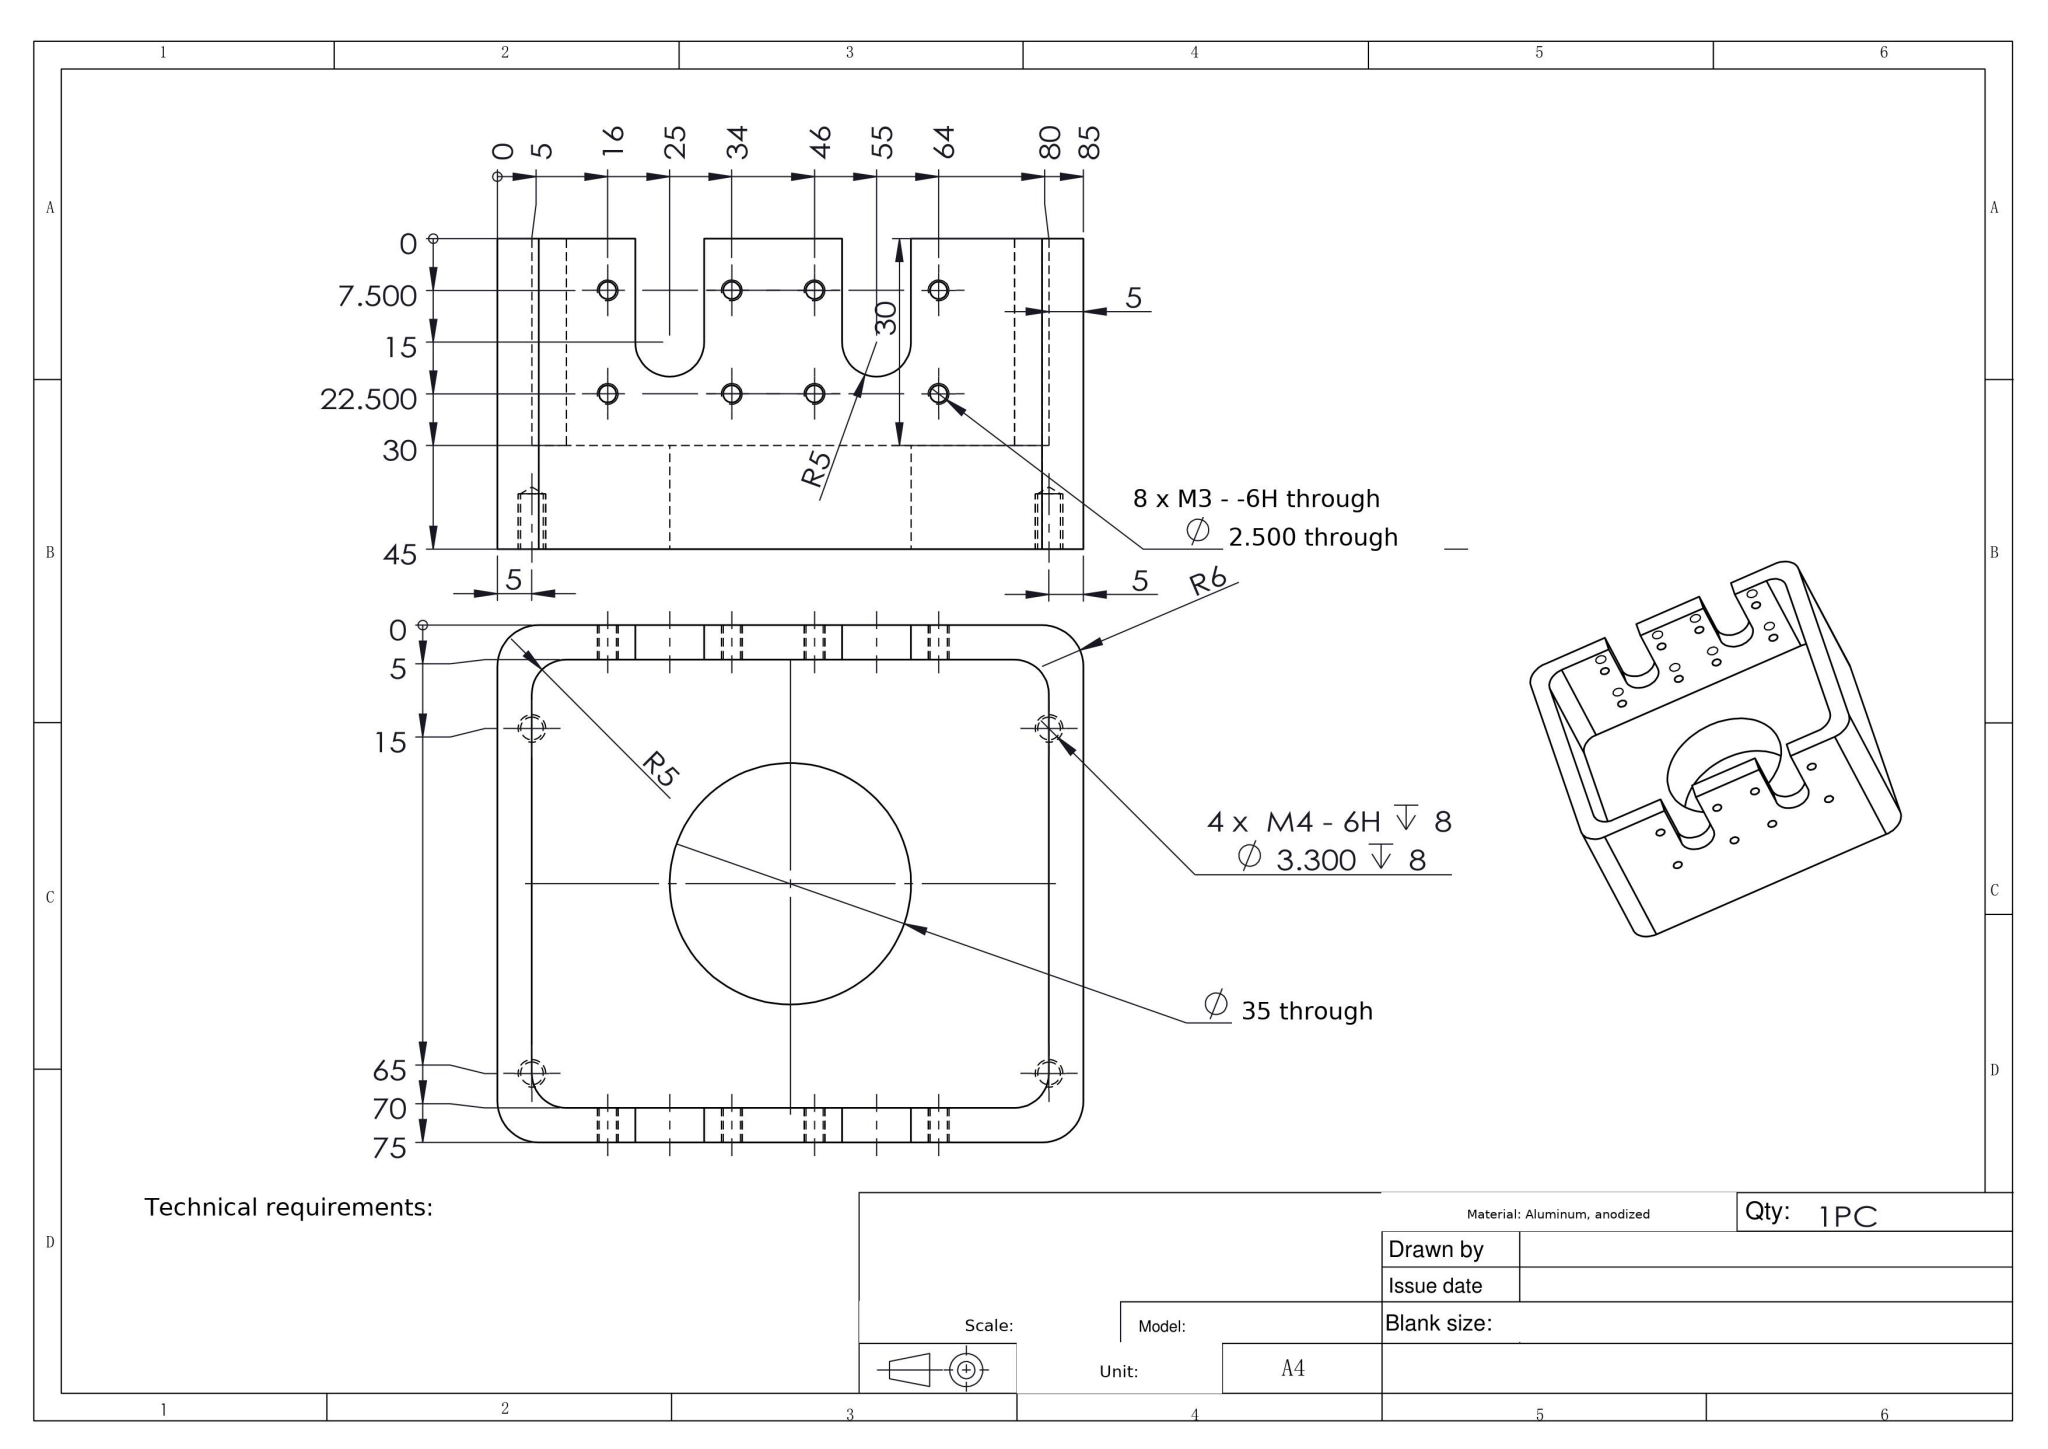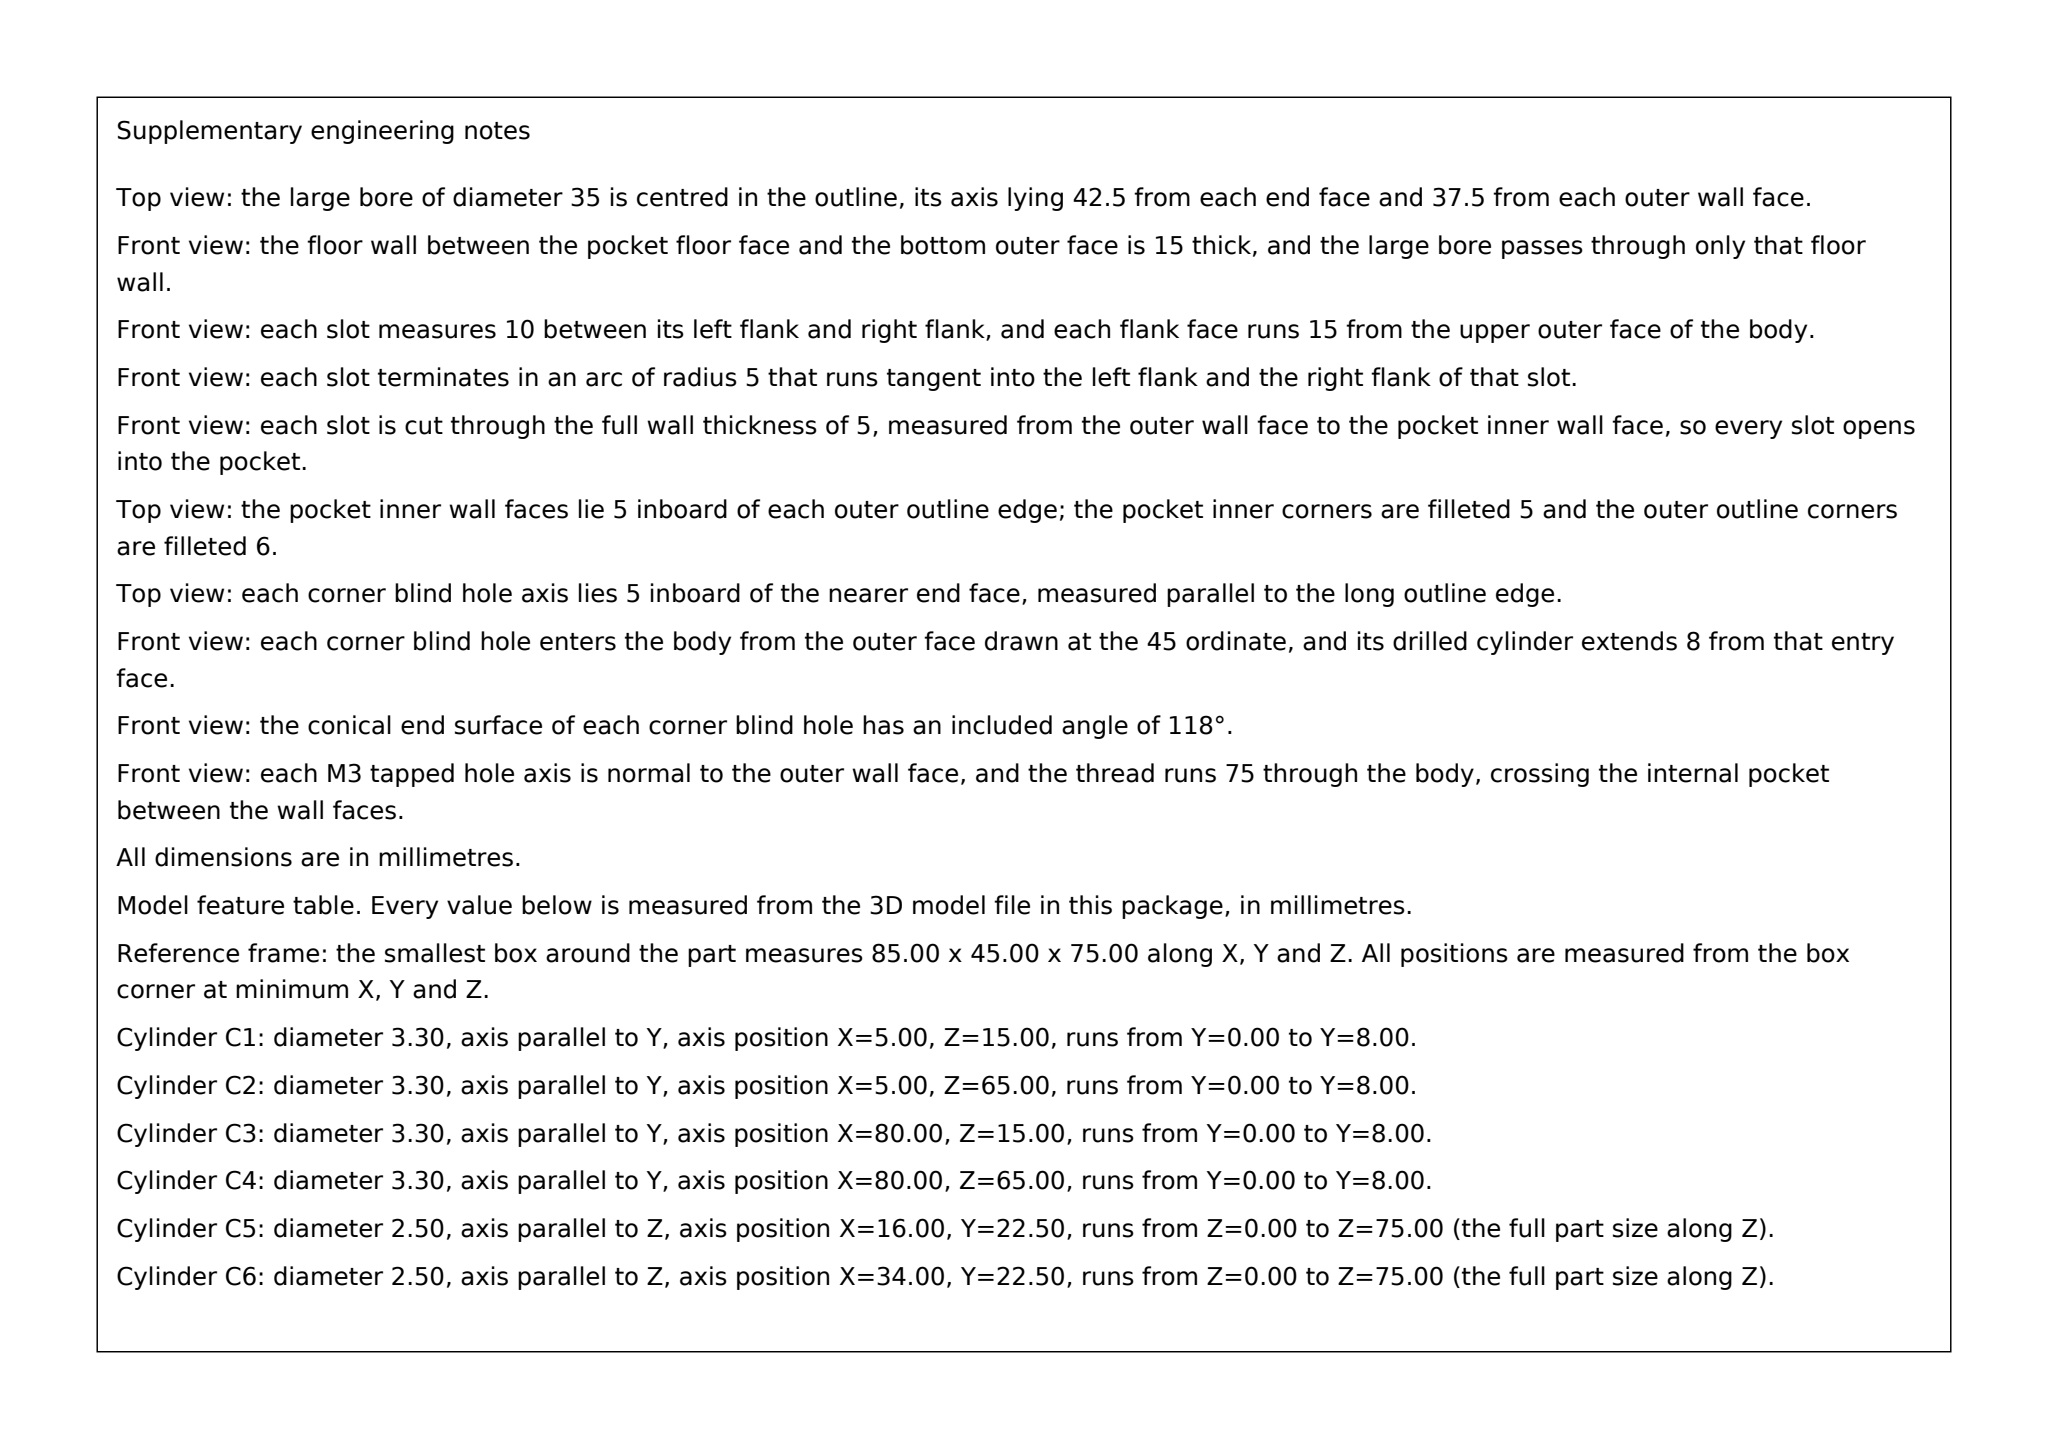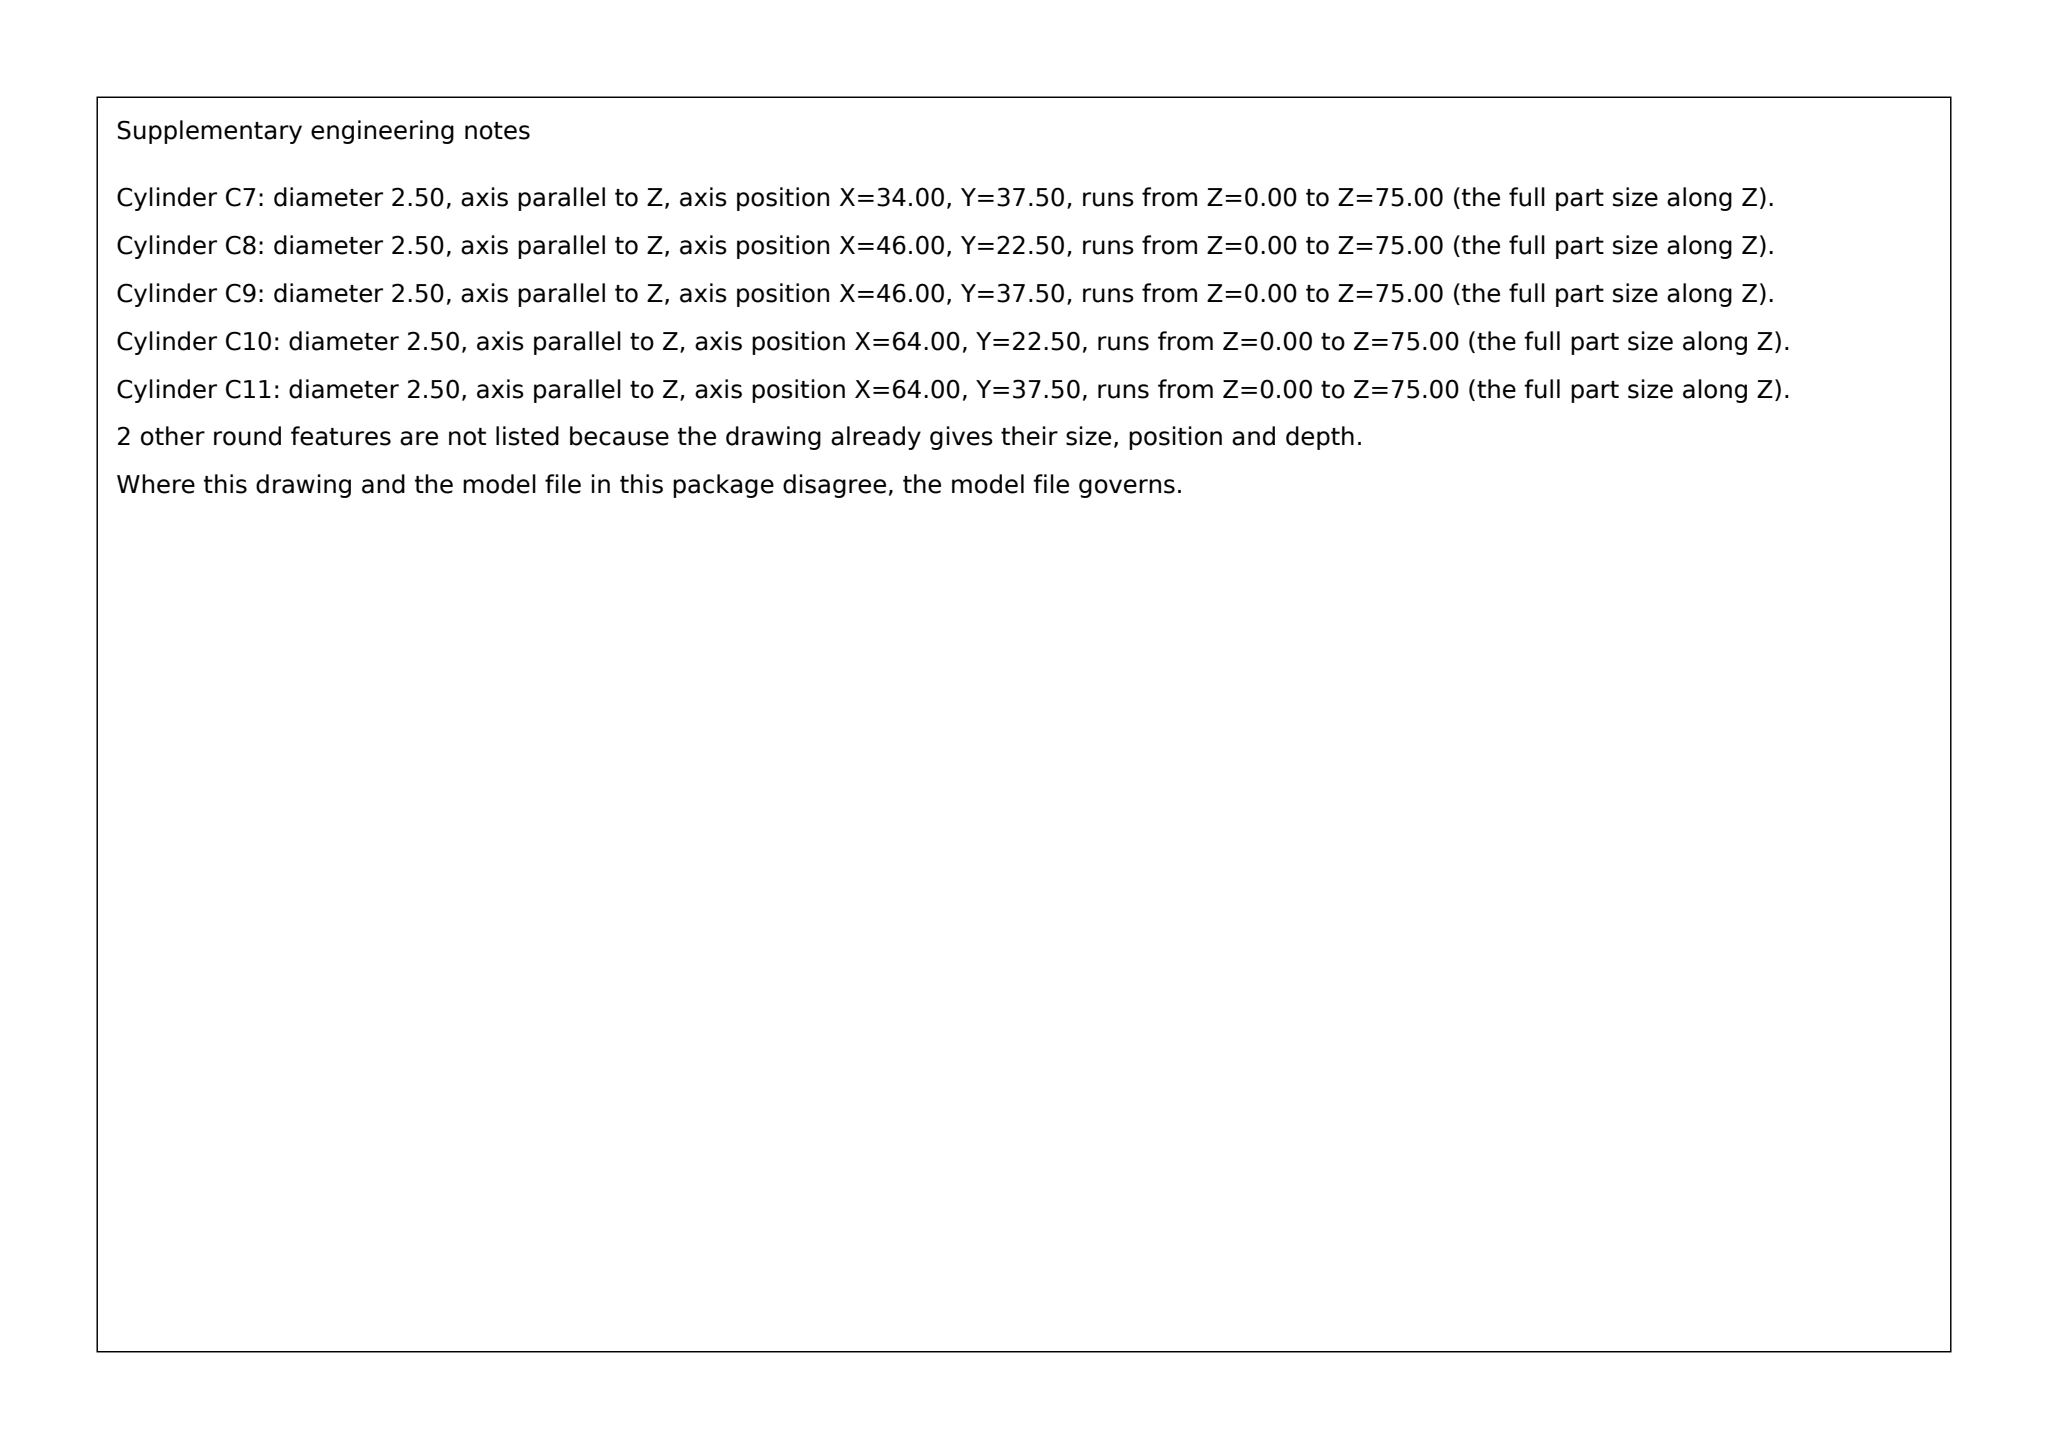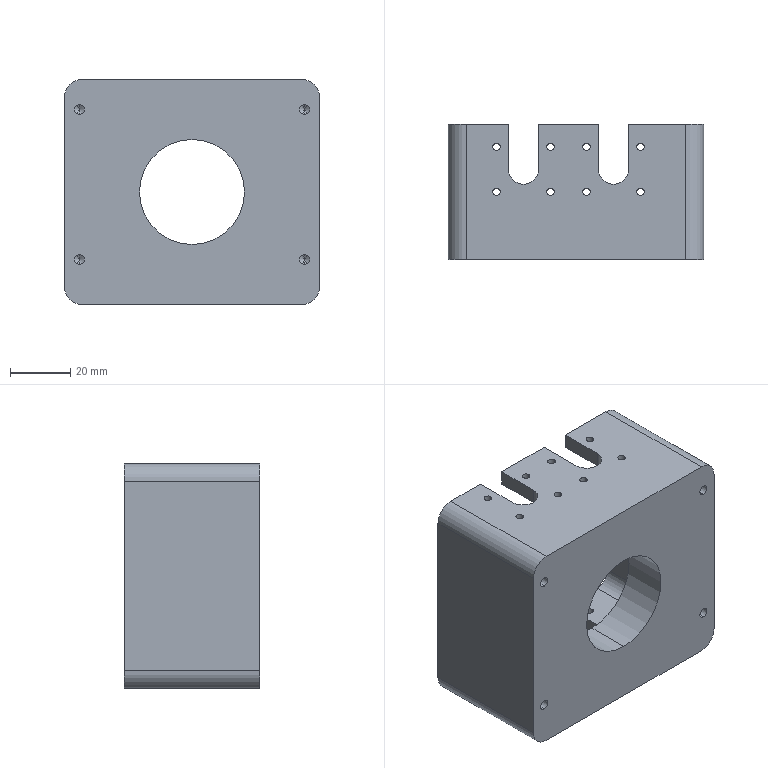Part | SolidWorks | mm | 1 solid | 84 faces | box 85 x 45 x 75 mm | volume 120983 mm3 | cylinder 54 | plane 22 | cone 8 | commonest cylinder face diameters 2.5 x32 3.3 x8 10 x8 12 x4 35 x2
Drawing notes:
SLOT AT X=25: 10 WIDE (WALLS X20/X30), R5 FULL RAD BOT, 15 DP FROM TOP FACE | from the solid: x-planes 20 & 30 (width 10); Ø10 z-axis cyl at x=25, y=30 (=15 below top face y=45), len 5 = wall thk
SLOT AT X=55: 10 WIDE (WALLS X50/X60), R5 FULL RAD BOT, 15 DP FROM TOP FACE | from the solid: x-planes 50 & 60 (width 10); Ø10 z-axis cyl at x=55, y=30, len 5 = wall thk
8 x M3 THRU IN EACH 5 THK WALL, FRONT & REAR - 16 TOTAL | from the solid: Ø2.5 z-axis holes at x=16/34/46/64, y=22.5 & 37.5, len 5, in walls z 0-5 and z 70-75
build123d program:
from build123d import *

# Parameters (mm, degrees)
SKETCH1_W             = 85
SKETCH1_H             = 75
BOSS_EXTRUDE1_DEPTH   = 45
SKETCH2_R             = 5
CUT_EXTRUDE1_DEPTH    = 122.963
M3_TAPPED_HOLE1_D     = 2.5
SKETCH5_W             = 10
SKETCH5_H             = 15
CUT_EXTRUDE2_DEPTH    = 80
LPATTERN1_COUNT       = 2
LPATTERN1_PITCH       = 30
SKETCH7_W             = 75
SKETCH7_H             = 65
CUT_EXTRUDE3_DEPTH    = 30
M4_TAPPED_HOLE1_D     = 3.3
M4_TAPPED_HOLE1_DEPTH = 8
M4_TAPPED_HOLE1_TIP   = 0.9914
FILLET1_R             = 5
SKETCH10_R            = 17.5
CUT_EXTRUDE4_DEPTH    = 118.26
FILLET2_R             = 6


with BuildPart() as part:
    # Sketch1 → Boss-Extrude1 (new body)
    with BuildSketch(Plane(origin=(0, 0, 0), x_dir=(1, 0, 0), z_dir=(0, 1, 0))):
        with Locations((42.5, 37.5)):
            Rectangle(SKETCH1_W, SKETCH1_H)
    extrude(amount=BOSS_EXTRUDE1_DEPTH)

    # Sketch2 → Cut-Extrude1 (cut, through all)
    with BuildSketch(Plane.XY):
        with Locations((25, 30)):
            Circle(SKETCH2_R)
        with Locations((55, 30)):
            Circle(SKETCH2_R)
    extrude(amount=-CUT_EXTRUDE1_DEPTH, mode=Mode.SUBTRACT)

    # M3 Tapped Hole1 (through all)
    with Locations(Plane.XY):
        with Locations((16, 37.5), (16, 22.5), (34, 22.5), (34, 37.5)):
            m3_tapped_hole1 = Hole(M3_TAPPED_HOLE1_D / 2)

    # Sketch5 → Cut-Extrude2 (cut)
    with BuildSketch(Plane.XY):
        with Locations((25, 37.5)):
            Rectangle(SKETCH5_W, SKETCH5_H)
    cut_extrude2 = extrude(amount=-CUT_EXTRUDE2_DEPTH, mode=Mode.SUBTRACT)

    # LPattern1: M3 Tapped Hole1, Cut-Extrude2 ×2
    with Locations(*[(i * LPATTERN1_PITCH, 0, 0) for i in range(1, LPATTERN1_COUNT)]):
        add(m3_tapped_hole1, mode=Mode.SUBTRACT)
        add(cut_extrude2, mode=Mode.SUBTRACT)

    # Sketch7 → Cut-Extrude3 (cut)
    with BuildSketch(Plane(origin=(0, 45, 0), x_dir=(1, 0, 0), z_dir=(0, 1, 0))):
        with Locations((42.5, 37.5)):
            Rectangle(SKETCH7_W, SKETCH7_H)
    extrude(amount=-CUT_EXTRUDE3_DEPTH, mode=Mode.SUBTRACT)

    # M4 Tapped Hole1
    with Locations(Plane(origin=(0, 0, 0), x_dir=(-1, 0, 0), z_dir=(0, -1, 0))):
        with Locations((-5, 60), (-5, 10), (-80, 10), (-80, 60)):
            Hole(M4_TAPPED_HOLE1_D / 2, depth=M4_TAPPED_HOLE1_DEPTH)
            with Locations((0, 0, -(M4_TAPPED_HOLE1_DEPTH + M4_TAPPED_HOLE1_TIP / 2))):  # 118° drill point
                Cone(0, M4_TAPPED_HOLE1_D / 2, M4_TAPPED_HOLE1_TIP, mode=Mode.SUBTRACT)

    # Fillet1
    fillet1_edges = [part.edges().sort_by_distance(p)[0] for p in [
        (5, 30, -70),
        (80, 30, -5),
        (5, 30, -5),
        (80, 30, -70),
    ]]
    fillet(fillet1_edges, radius=FILLET1_R)

    # Sketch10 → Cut-Extrude4 (cut, through all)
    with BuildSketch(Plane(origin=(0, 15, 0), x_dir=(1, 0, 0), z_dir=(0, 1, 0))):
        with Locations(Location((42.5, 37.5, 0), (0, 0, 270))):
            Circle(SKETCH10_R)
    extrude(amount=-CUT_EXTRUDE4_DEPTH, mode=Mode.SUBTRACT)

    # Fillet2
    fillet2_edges = [part.edges().sort_by_distance(p)[0] for p in [
        (0, 22.5, -75),
        (85, 22.5, -75),
        (85, 22.5, 0),
        (0, 22.5, 0),
    ]]
    fillet(fillet2_edges, radius=FILLET2_R)


solid = part.part